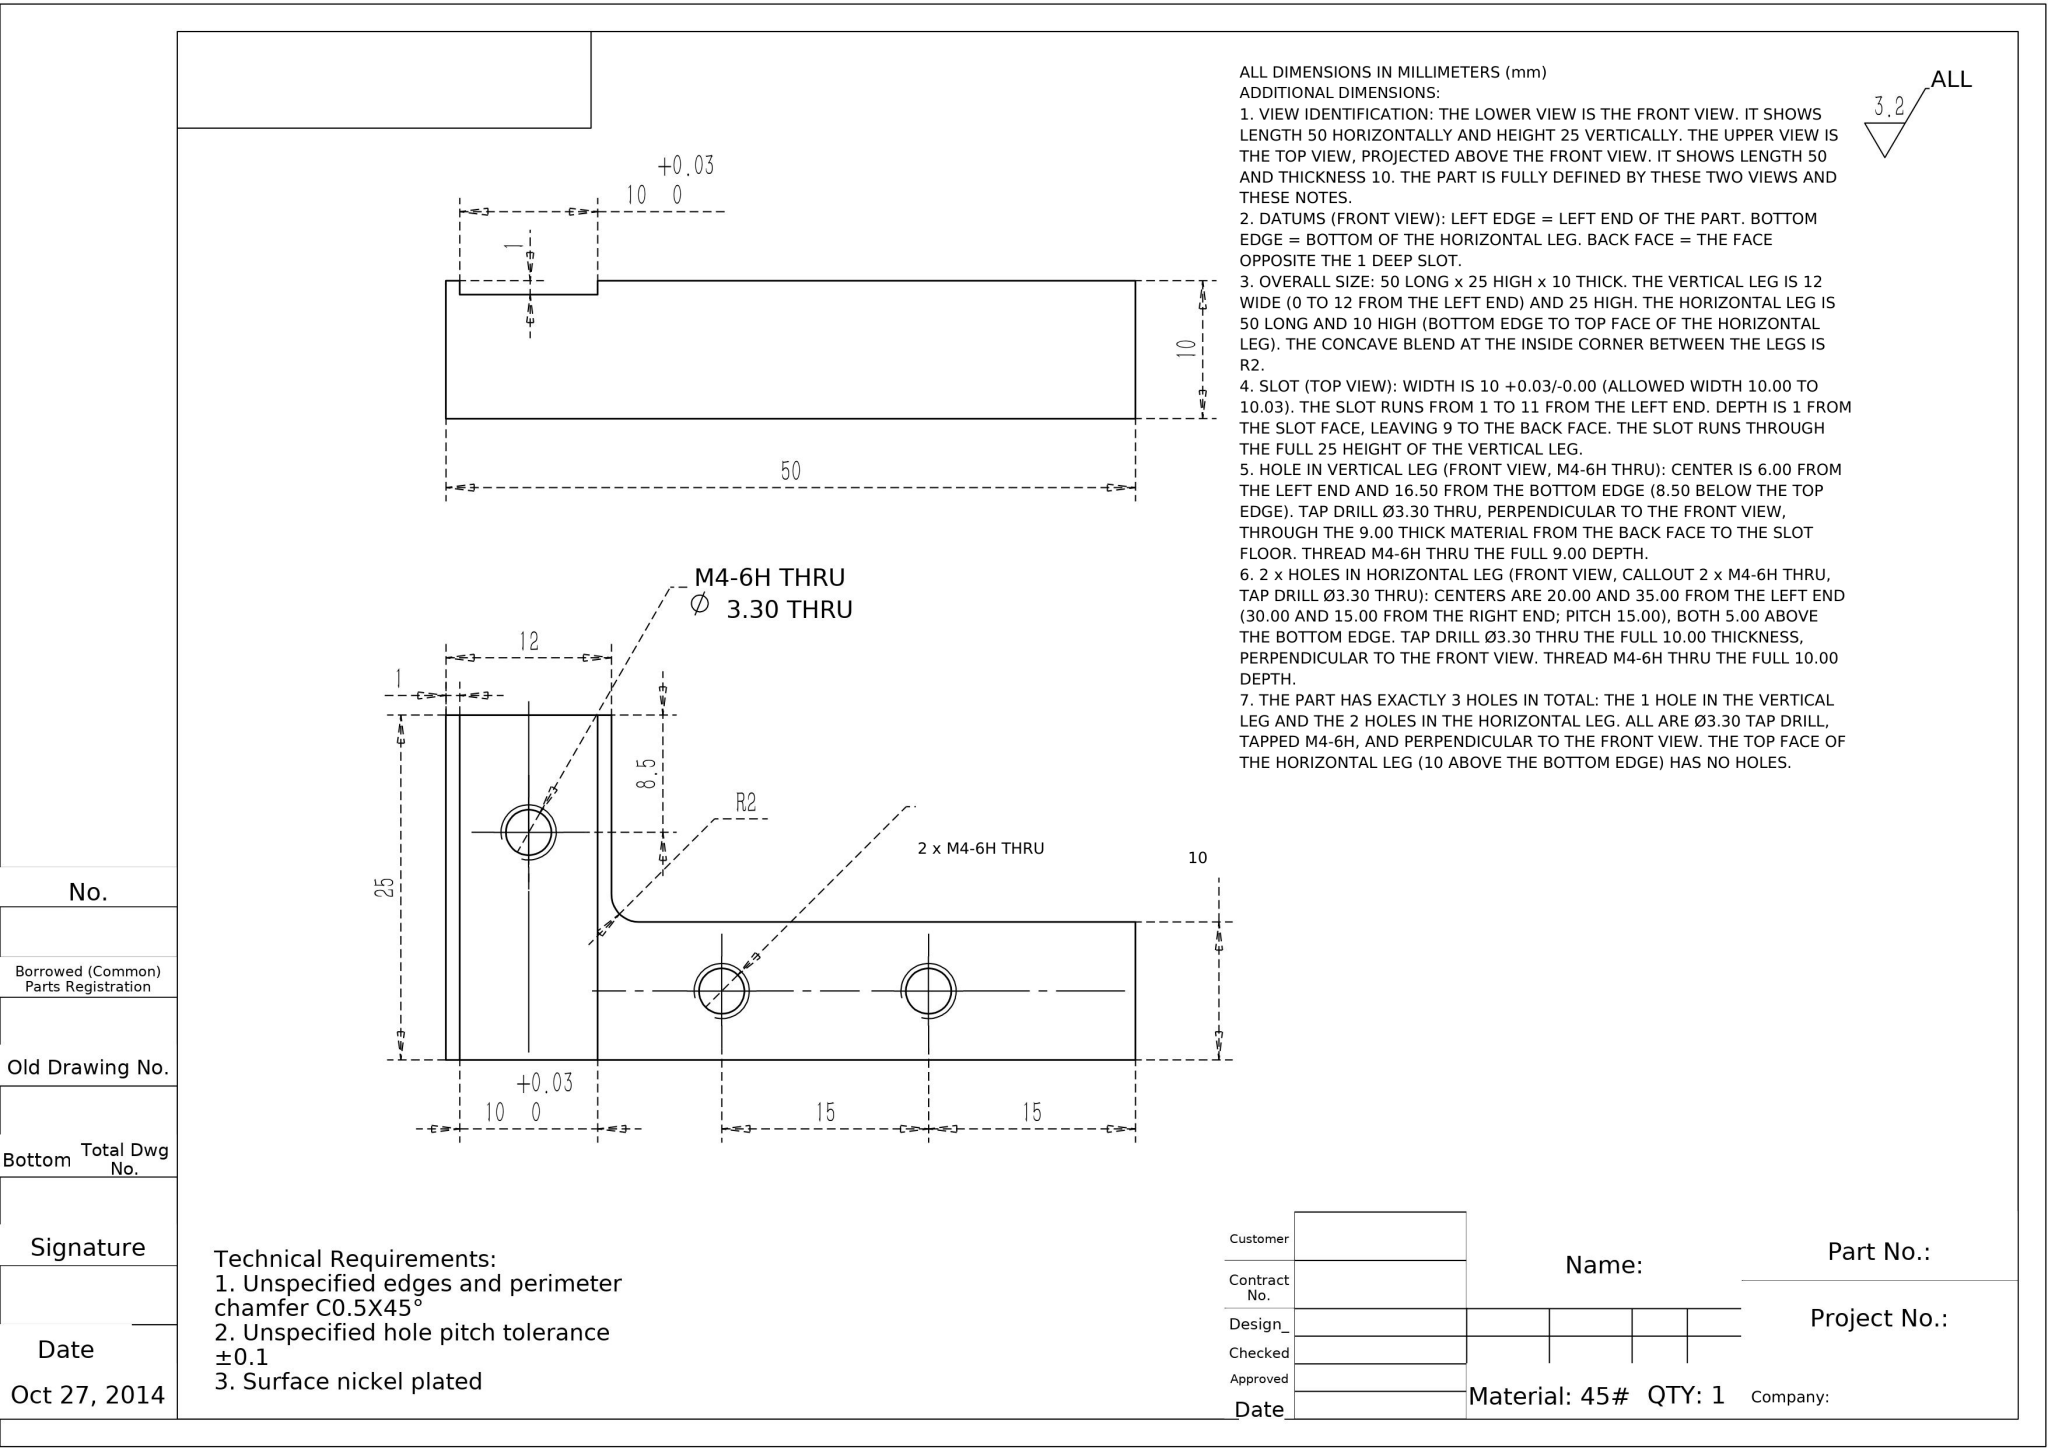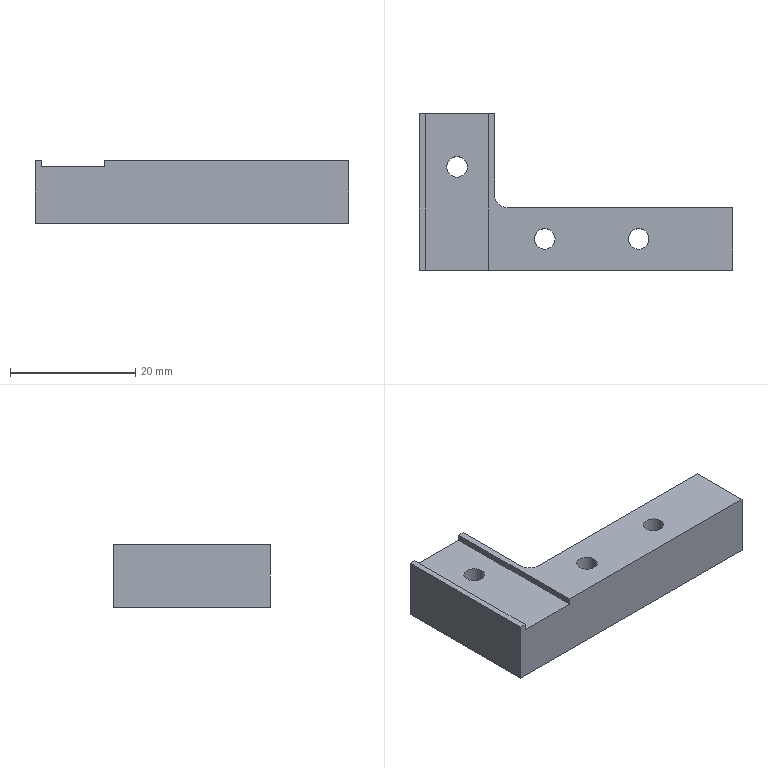Part | NX | mm | L-Shaped Three-Bore Mounting Bracket 50mm | 1 solid | 19 faces | box 50 x 25 x 10 mm | volume 6311 mm3 | plane 12 | cylinder 7 | commonest cylinder face diameters 3.3 x6 4 x1